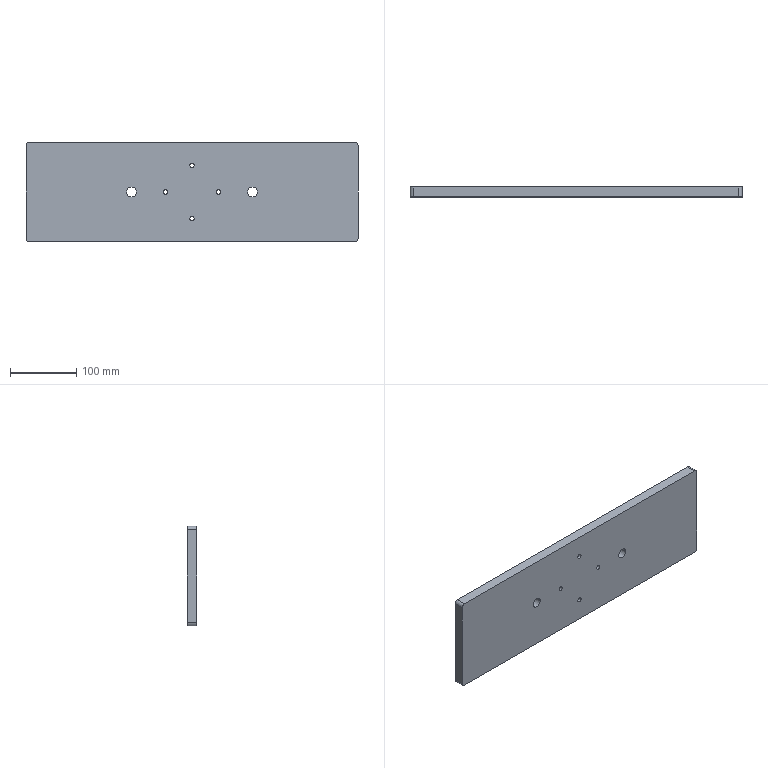Component | SolidWorks | E006TopPlate-1 | 1 solid | 22 faces | box 500 x 15 x 150 mm | volume 1117198 mm3 | cylinder 16 | plane 6 | commonest cylinder face diameters 6.8 x8 15 x4 10 x4 | material Plain Carbon Steel
build123d program:
from build123d import *

# Parameters (mm, degrees)
SKETCH1_W           = 500
SKETCH1_H           = 150
BOSS_EXTRUDE1_DEPTH = 7.5
FILLET1_R           = 5
SKETCH7_R           = 7.5
CUT_EXTRUDE2_DEPTH  = 262.438
M8_TAPPED_HOLE1_D   = 6.8


with BuildPart() as part:
    # Sketch1 → Boss-Extrude1 (new, symmetric)
    with BuildSketch(Plane.XY):
        Rectangle(SKETCH1_W, SKETCH1_H)
    extrude(amount=BOSS_EXTRUDE1_DEPTH, both=True)

    # Fillet1
    fillet1_edges = [part.edges().sort_by_distance(p)[0] for p in [
        (250, -75, 0),
        (-250, -75, 0),
        (-250, 75, 0),
        (250, 75, 0),
    ]]
    fillet(fillet1_edges, radius=FILLET1_R)

    # Sketch7 → Cut-Extrude2 (cut, through all)
    with BuildSketch(Plane.XY.offset(7.5)):
        with Locations((-91, 0)):
            Circle(SKETCH7_R)
    cut_extrude2 = extrude(amount=-CUT_EXTRUDE2_DEPTH, mode=Mode.SUBTRACT)

    # M8 Tapped Hole1 (through all)
    with Locations(Plane.XY.offset(7.5)):
        with Locations((0, 40), (0, -40), (-40, 0), (40, 0)):
            Hole(M8_TAPPED_HOLE1_D / 2)

    # Mirror1: Cut-Extrude2 across plane
    add(cut_extrude2.mirror(Plane(origin=(0, 0, 0), x_dir=(0, 0, 1), z_dir=(1, 0, 0))), mode=Mode.SUBTRACT)


solid = part.part

# Placed as in the assembly
solid = solid.moved(Location((0, 288.5, 0), (90, 0, 0)))
STEP:
#1=COLOUR_RGB('',0.7922,0.8196,0.9333);
#2=FILL_AREA_STYLE_COLOUR('',#1);
#3=FILL_AREA_STYLE('',(#2));
#4=SURFACE_STYLE_FILL_AREA(#3);
#5=SURFACE_SIDE_STYLE('',(#4));
#6=SURFACE_STYLE_USAGE(.BOTH.,#5);
#7=PRESENTATION_STYLE_ASSIGNMENT((#6));
#8=CARTESIAN_POINT('',(3.878,11.063,-0.));
#9=VERTEX_POINT('',#8);
#10=CARTESIAN_POINT('',(3.287,11.063,-0.));
#11=VERTEX_POINT('',#10);
#12=CARTESIAN_POINT('',(3.583,11.063,-0.));
#13=DIRECTION('',(0.,-1.,0.));
#14=DIRECTION('',(-1.,0.,0.));
#15=AXIS2_PLACEMENT_3D('',#12,#13,#14);
#16=CIRCLE('',#15,0.2953);
#17=EDGE_CURVE('',#9,#11,#16,.T.);
#18=ORIENTED_EDGE('',*,*,#17,.T.);
#19=CARTESIAN_POINT('',(3.287,11.654,-0.));
#20=VERTEX_POINT('',#19);
#21=CARTESIAN_POINT('',(3.287,11.063,-0.));
#22=DIRECTION('',(0.,1.,0.));
#23=VECTOR('',#22,39.37);
#24=LINE('',#21,#23);
#25=EDGE_CURVE('',#11,#20,#24,.T.);
#26=ORIENTED_EDGE('',*,*,#25,.T.);
#27=CARTESIAN_POINT('',(3.878,11.654,-0.));
#28=VERTEX_POINT('',#27);
#29=CARTESIAN_POINT('',(3.583,11.654,-0.));
#30=DIRECTION('',(0.,-1.,0.));
#31=DIRECTION('',(-1.,0.,0.));
#32=AXIS2_PLACEMENT_3D('',#29,#30,#31);
#33=CIRCLE('',#32,0.2953);
#34=EDGE_CURVE('',#28,#20,#33,.T.);
#35=ORIENTED_EDGE('',*,*,#34,.F.);
#36=CARTESIAN_POINT('',(3.878,11.063,-0.));
#37=DIRECTION('',(0.,1.,0.));
#38=VECTOR('',#37,39.37);
#39=LINE('',#36,#38);
#40=EDGE_CURVE('',#9,#28,#39,.T.);
#41=ORIENTED_EDGE('',*,*,#40,.F.);
#42=EDGE_LOOP('',(#18,#26,#35,#41));
#43=FACE_OUTER_BOUND('',#42,.T.);
#44=CARTESIAN_POINT('',(3.583,11.063,-0.));
#45=DIRECTION('',(0.,1.,0.));
#46=DIRECTION('',(1.,0.,-0.));
#47=AXIS2_PLACEMENT_3D('',#44,#45,#46);
#48=CYLINDRICAL_SURFACE('',#47,0.2953);
#49=ADVANCED_FACE('',(#43),#48,.F.);
#50=CARTESIAN_POINT('',(-0.1339,11.063,-1.575));
#51=VERTEX_POINT('',#50);
#52=CARTESIAN_POINT('',(0.1339,11.063,-1.575));
#53=VERTEX_POINT('',#52);
#54=CARTESIAN_POINT('',(-0.,11.063,-1.575));
#55=DIRECTION('',(0.,1.,0.));
#56=DIRECTION('',(1.,0.,0.));
#57=AXIS2_PLACEMENT_3D('',#54,#55,#56);
#58=CIRCLE('',#57,0.1339);
#59=EDGE_CURVE('',#51,#53,#58,.T.);
#60=ORIENTED_EDGE('',*,*,#59,.F.);
#61=CARTESIAN_POINT('',(-0.1339,11.654,-1.575));
#62=VERTEX_POINT('',#61);
#63=CARTESIAN_POINT('',(-0.1339,11.654,-1.575));
#64=DIRECTION('',(0.,1.,0.));
#65=VECTOR('',#64,39.37);
#66=LINE('',#63,#65);
#67=EDGE_CURVE('',#51,#62,#66,.T.);
#68=ORIENTED_EDGE('',*,*,#67,.T.);
#69=CARTESIAN_POINT('',(0.1339,11.654,-1.575));
#70=VERTEX_POINT('',#69);
#71=CARTESIAN_POINT('',(-0.,11.654,-1.575));
#72=DIRECTION('',(0.,1.,0.));
#73=DIRECTION('',(1.,0.,0.));
#74=AXIS2_PLACEMENT_3D('',#71,#72,#73);
#75=CIRCLE('',#74,0.1339);
#76=EDGE_CURVE('',#62,#70,#75,.T.);
#77=ORIENTED_EDGE('',*,*,#76,.T.);
#78=CARTESIAN_POINT('',(0.1339,11.654,-1.575));
#79=DIRECTION('',(0.,1.,0.));
#80=VECTOR('',#79,39.37);
#81=LINE('',#78,#80);
#82=EDGE_CURVE('',#53,#70,#81,.T.);
#83=ORIENTED_EDGE('',*,*,#82,.F.);
#84=EDGE_LOOP('',(#60,#68,#77,#83));
#85=FACE_OUTER_BOUND('',#84,.T.);
#86=CARTESIAN_POINT('',(-0.,11.654,-1.575));
#87=DIRECTION('',(0.,1.,0.));
#88=DIRECTION('',(1.,0.,0.));
#89=AXIS2_PLACEMENT_3D('',#86,#87,#88);
#90=CYLINDRICAL_SURFACE('',#89,0.1339);
#91=ADVANCED_FACE('',(#85),#90,.F.);
#92=CARTESIAN_POINT('',(-0.1339,11.063,1.575));
#93=VERTEX_POINT('',#92);
#94=CARTESIAN_POINT('',(0.1339,11.063,1.575));
#95=VERTEX_POINT('',#94);
#96=CARTESIAN_POINT('',(-0.,11.063,1.575));
#97=DIRECTION('',(0.,1.,0.));
#98=DIRECTION('',(1.,0.,0.));
#99=AXIS2_PLACEMENT_3D('',#96,#97,#98);
#100=CIRCLE('',#99,0.1339);
#101=EDGE_CURVE('',#93,#95,#100,.T.);
#102=ORIENTED_EDGE('',*,*,#101,.F.);
#103=CARTESIAN_POINT('',(-0.1339,11.654,1.575));
#104=VERTEX_POINT('',#103);
#105=CARTESIAN_POINT('',(-0.1339,11.654,1.575));
#106=DIRECTION('',(0.,1.,0.));
#107=VECTOR('',#106,39.37);
#108=LINE('',#105,#107);
#109=EDGE_CURVE('',#93,#104,#108,.T.);
#110=ORIENTED_EDGE('',*,*,#109,.T.);
#111=CARTESIAN_POINT('',(0.1339,11.654,1.575));
#112=VERTEX_POINT('',#111);
#113=CARTESIAN_POINT('',(-0.,11.654,1.575));
#114=DIRECTION('',(0.,1.,0.));
#115=DIRECTION('',(1.,0.,0.));
#116=AXIS2_PLACEMENT_3D('',#113,#114,#115);
#117=CIRCLE('',#116,0.1339);
#118=EDGE_CURVE('',#104,#112,#117,.T.);
#119=ORIENTED_EDGE('',*,*,#118,.T.);
#120=CARTESIAN_POINT('',(0.1339,11.654,1.575));
#121=DIRECTION('',(0.,1.,0.));
#122=VECTOR('',#121,39.37);
#123=LINE('',#120,#122);
#124=EDGE_CURVE('',#95,#112,#123,.T.);
#125=ORIENTED_EDGE('',*,*,#124,.F.);
#126=EDGE_LOOP('',(#102,#110,#119,#125));
#127=FACE_OUTER_BOUND('',#126,.T.);
#128=CARTESIAN_POINT('',(-0.,11.654,1.575));
#129=DIRECTION('',(0.,1.,0.));
#130=DIRECTION('',(1.,0.,0.));
#131=AXIS2_PLACEMENT_3D('',#128,#129,#130);
#132=CYLINDRICAL_SURFACE('',#131,0.1339);
#133=ADVANCED_FACE('',(#127),#132,.F.);
#134=CARTESIAN_POINT('',(-1.709,11.063,0.));
#135=VERTEX_POINT('',#134);
#136=CARTESIAN_POINT('',(-1.441,11.063,0.));
#137=VERTEX_POINT('',#136);
#138=CARTESIAN_POINT('',(-1.575,11.063,0.));
#139=DIRECTION('',(0.,1.,0.));
#140=DIRECTION('',(1.,0.,-0.));
#141=AXIS2_PLACEMENT_3D('',#138,#139,#140);
#142=CIRCLE('',#141,0.1339);
#143=EDGE_CURVE('',#135,#137,#142,.T.);
#144=ORIENTED_EDGE('',*,*,#143,.F.);
#145=CARTESIAN_POINT('',(-1.709,11.654,0.));
#146=VERTEX_POINT('',#145);
#147=CARTESIAN_POINT('',(-1.709,11.654,0.));
#148=DIRECTION('',(0.,1.,0.));
#149=VECTOR('',#148,39.37);
#150=LINE('',#147,#149);
#151=EDGE_CURVE('',#135,#146,#150,.T.);
#152=ORIENTED_EDGE('',*,*,#151,.T.);
#153=CARTESIAN_POINT('',(-1.441,11.654,0.));
#154=VERTEX_POINT('',#153);
#155=CARTESIAN_POINT('',(-1.575,11.654,0.));
#156=DIRECTION('',(0.,1.,0.));
#157=DIRECTION('',(1.,0.,-0.));
#158=AXIS2_PLACEMENT_3D('',#155,#156,#157);
#159=CIRCLE('',#158,0.1339);
#160=EDGE_CURVE('',#146,#154,#159,.T.);
#161=ORIENTED_EDGE('',*,*,#160,.T.);
#162=CARTESIAN_POINT('',(-1.441,11.654,0.));
#163=DIRECTION('',(0.,1.,0.));
#164=VECTOR('',#163,39.37);
#165=LINE('',#162,#164);
#166=EDGE_CURVE('',#137,#154,#165,.T.);
#167=ORIENTED_EDGE('',*,*,#166,.F.);
#168=EDGE_LOOP('',(#144,#152,#161,#167));
#169=FACE_OUTER_BOUND('',#168,.T.);
#170=CARTESIAN_POINT('',(-1.575,11.654,0.));
#171=DIRECTION('',(0.,1.,0.));
#172=DIRECTION('',(1.,0.,-0.));
#173=AXIS2_PLACEMENT_3D('',#170,#171,#172);
#174=CYLINDRICAL_SURFACE('',#173,0.1339);
#175=ADVANCED_FACE('',(#169),#174,.F.);
#176=CARTESIAN_POINT('',(1.441,11.063,-0.));
#177=VERTEX_POINT('',#176);
#178=CARTESIAN_POINT('',(1.709,11.063,0.));
#179=VERTEX_POINT('',#178);
#180=CARTESIAN_POINT('',(1.575,11.063,0.));
#181=DIRECTION('',(0.,1.,0.));
#182=DIRECTION('',(1.,0.,-0.));
#183=AXIS2_PLACEMENT_3D('',#180,#181,#182);
#184=CIRCLE('',#183,0.1339);
#185=EDGE_CURVE('',#177,#179,#184,.T.);
#186=ORIENTED_EDGE('',*,*,#185,.F.);
#187=CARTESIAN_POINT('',(1.441,11.654,-0.));
#188=VERTEX_POINT('',#187);
#189=CARTESIAN_POINT('',(1.441,11.654,-0.));
#190=DIRECTION('',(0.,1.,0.));
#191=VECTOR('',#190,39.37);
#192=LINE('',#189,#191);
#193=EDGE_CURVE('',#177,#188,#192,.T.);
#194=ORIENTED_EDGE('',*,*,#193,.T.);
#195=CARTESIAN_POINT('',(1.709,11.654,0.));
#196=VERTEX_POINT('',#195);
#197=CARTESIAN_POINT('',(1.575,11.654,0.));
#198=DIRECTION('',(0.,1.,0.));
#199=DIRECTION('',(1.,0.,-0.));
#200=AXIS2_PLACEMENT_3D('',#197,#198,#199);
#201=CIRCLE('',#200,0.1339);
#202=EDGE_CURVE('',#188,#196,#201,.T.);
#203=ORIENTED_EDGE('',*,*,#202,.T.);
#204=CARTESIAN_POINT('',(1.709,11.654,0.));
#205=DIRECTION('',(0.,1.,0.));
#206=VECTOR('',#205,39.37);
#207=LINE('',#204,#206);
#208=EDGE_CURVE('',#179,#196,#207,.T.);
#209=ORIENTED_EDGE('',*,*,#208,.F.);
#210=EDGE_LOOP('',(#186,#194,#203,#209));
#211=FACE_OUTER_BOUND('',#210,.T.);
#212=CARTESIAN_POINT('',(1.575,11.654,0.));
#213=DIRECTION('',(0.,1.,0.));
#214=DIRECTION('',(1.,0.,-0.));
#215=AXIS2_PLACEMENT_3D('',#212,#213,#214);
#216=CYLINDRICAL_SURFACE('',#215,0.1339);
#217=ADVANCED_FACE('',(#211),#216,.F.);
#218=CARTESIAN_POINT('',(-3.878,11.063,0.));
#219=VERTEX_POINT('',#218);
#220=CARTESIAN_POINT('',(-3.287,11.063,0.));
#221=VERTEX_POINT('',#220);
#222=CARTESIAN_POINT('',(-3.583,11.063,0.));
#223=DIRECTION('',(0.,1.,0.));
#224=DIRECTION('',(1.,0.,-0.));
#225=AXIS2_PLACEMENT_3D('',#222,#223,#224);
#226=CIRCLE('',#225,0.2953);
#227=EDGE_CURVE('',#219,#221,#226,.T.);
#228=ORIENTED_EDGE('',*,*,#227,.F.);
#229=CARTESIAN_POINT('',(-3.878,11.654,0.));
#230=VERTEX_POINT('',#229);
#231=CARTESIAN_POINT('',(-3.878,11.063,0.));
#232=DIRECTION('',(0.,1.,0.));
#233=VECTOR('',#232,39.37);
#234=LINE('',#231,#233);
#235=EDGE_CURVE('',#219,#230,#234,.T.);
#236=ORIENTED_EDGE('',*,*,#235,.T.);
#237=CARTESIAN_POINT('',(-3.287,11.654,0.));
#238=VERTEX_POINT('',#237);
#239=CARTESIAN_POINT('',(-3.583,11.654,0.));
#240=DIRECTION('',(0.,1.,0.));
#241=DIRECTION('',(1.,0.,-0.));
#242=AXIS2_PLACEMENT_3D('',#239,#240,#241);
#243=CIRCLE('',#242,0.2953);
#244=EDGE_CURVE('',#230,#238,#243,.T.);
#245=ORIENTED_EDGE('',*,*,#244,.T.);
#246=CARTESIAN_POINT('',(-3.287,11.063,0.));
#247=DIRECTION('',(0.,1.,0.));
#248=VECTOR('',#247,39.37);
#249=LINE('',#246,#248);
#250=EDGE_CURVE('',#221,#238,#249,.T.);
#251=ORIENTED_EDGE('',*,*,#250,.F.);
#252=EDGE_LOOP('',(#228,#236,#245,#251));
#253=FACE_OUTER_BOUND('',#252,.T.);
#254=CARTESIAN_POINT('',(-3.583,11.063,0.));
#255=DIRECTION('',(0.,1.,0.));
#256=DIRECTION('',(1.,0.,-0.));
#257=AXIS2_PLACEMENT_3D('',#254,#255,#256);
#258=CYLINDRICAL_SURFACE('',#257,0.2953);
#259=ADVANCED_FACE('',(#253),#258,.F.);
#260=CARTESIAN_POINT('',(-9.646,11.654,2.953));
#261=VERTEX_POINT('',#260);
#262=CARTESIAN_POINT('',(9.646,11.654,2.953));
#263=VERTEX_POINT('',#262);
#264=CARTESIAN_POINT('',(-9.843,11.654,2.953));
#265=DIRECTION('',(1.,0.,-0.));
#266=VECTOR('',#265,39.37);
#267=LINE('',#264,#266);
#268=EDGE_CURVE('',#261,#263,#267,.T.);
#269=ORIENTED_EDGE('',*,*,#268,.T.);
#270=CARTESIAN_POINT('',(9.843,11.654,2.756));
#271=VERTEX_POINT('',#270);
#272=CARTESIAN_POINT('',(9.646,11.654,2.756));
#273=DIRECTION('',(0.,1.,0.));
#274=DIRECTION('',(1.,0.,0.));
#275=AXIS2_PLACEMENT_3D('',#272,#273,#274);
#276=CIRCLE('',#275,0.1969);
#277=EDGE_CURVE('',#263,#271,#276,.T.);
#278=ORIENTED_EDGE('',*,*,#277,.T.);
#279=CARTESIAN_POINT('',(9.843,11.654,-2.756));
#280=VERTEX_POINT('',#279);
#281=CARTESIAN_POINT('',(9.843,11.654,-2.953));
#282=DIRECTION('',(-0.,0.,-1.));
#283=VECTOR('',#282,39.37);
#284=LINE('',#281,#283);
#285=EDGE_CURVE('',#271,#280,#284,.T.);
#286=ORIENTED_EDGE('',*,*,#285,.T.);
#287=CARTESIAN_POINT('',(9.646,11.654,-2.953));
#288=VERTEX_POINT('',#287);
#289=CARTESIAN_POINT('',(9.646,11.654,-2.756));
#290=DIRECTION('',(0.,1.,0.));
#291=DIRECTION('',(1.,0.,0.));
#292=AXIS2_PLACEMENT_3D('',#289,#290,#291);
#293=CIRCLE('',#292,0.1969);
#294=EDGE_CURVE('',#280,#288,#293,.T.);
#295=ORIENTED_EDGE('',*,*,#294,.T.);
#296=CARTESIAN_POINT('',(-9.646,11.654,-2.953));
#297=VERTEX_POINT('',#296);
#298=CARTESIAN_POINT('',(-9.843,11.654,-2.953));
#299=DIRECTION('',(-1.,0.,0.));
#300=VECTOR('',#299,39.37);
#301=LINE('',#298,#300);
#302=EDGE_CURVE('',#288,#297,#301,.T.);
#303=ORIENTED_EDGE('',*,*,#302,.T.);
#304=CARTESIAN_POINT('',(-9.843,11.654,-2.756));
#305=VERTEX_POINT('',#304);
#306=CARTESIAN_POINT('',(-9.646,11.654,-2.756));
#307=DIRECTION('',(0.,1.,0.));
#308=DIRECTION('',(1.,0.,0.));
#309=AXIS2_PLACEMENT_3D('',#306,#307,#308);
#310=CIRCLE('',#309,0.1969);
#311=EDGE_CURVE('',#297,#305,#310,.T.);
#312=ORIENTED_EDGE('',*,*,#311,.T.);
#313=CARTESIAN_POINT('',(-9.843,11.654,2.756));
#314=VERTEX_POINT('',#313);
#315=CARTESIAN_POINT('',(-9.843,11.654,-2.953));
#316=DIRECTION('',(0.,0.,1.));
#317=VECTOR('',#316,39.37);
#318=LINE('',#315,#317);
#319=EDGE_CURVE('',#305,#314,#318,.T.);
#320=ORIENTED_EDGE('',*,*,#319,.T.);
#321=CARTESIAN_POINT('',(-9.646,11.654,2.756));
#322=DIRECTION('',(0.,1.,0.));
#323=DIRECTION('',(1.,0.,0.));
#324=AXIS2_PLACEMENT_3D('',#321,#322,#323);
#325=CIRCLE('',#324,0.1969);
#326=EDGE_CURVE('',#314,#261,#325,.T.);
#327=ORIENTED_EDGE('',*,*,#326,.T.);
#328=EDGE_LOOP('',(#269,#278,#286,#295,#303,#312,#320,#327));
#329=FACE_OUTER_BOUND('',#328,.T.);
#330=CARTESIAN_POINT('',(-3.583,11.654,0.));
#331=DIRECTION('',(0.,1.,0.));
#332=DIRECTION('',(1.,0.,-0.));
#333=AXIS2_PLACEMENT_3D('',#330,#331,#332);
#334=CIRCLE('',#333,0.2953);
#335=EDGE_CURVE('',#238,#230,#334,.T.);
#336=ORIENTED_EDGE('',*,*,#335,.F.);
#337=ORIENTED_EDGE('',*,*,#244,.F.);
#338=EDGE_LOOP('',(#336,#337));
#339=FACE_BOUND('',#338,.T.);
#340=CARTESIAN_POINT('',(1.575,11.654,0.));
#341=DIRECTION('',(0.,1.,0.));
#342=DIRECTION('',(1.,0.,-0.));
#343=AXIS2_PLACEMENT_3D('',#340,#341,#342);
#344=CIRCLE('',#343,0.1339);
#345=EDGE_CURVE('',#196,#188,#344,.T.);
#346=ORIENTED_EDGE('',*,*,#345,.F.);
#347=ORIENTED_EDGE('',*,*,#202,.F.);
#348=EDGE_LOOP('',(#346,#347));
#349=FACE_BOUND('',#348,.T.);
#350=CARTESIAN_POINT('',(-1.575,11.654,0.));
#351=DIRECTION('',(0.,1.,0.));
#352=DIRECTION('',(1.,0.,-0.));
#353=AXIS2_PLACEMENT_3D('',#350,#351,#352);
#354=CIRCLE('',#353,0.1339);
#355=EDGE_CURVE('',#154,#146,#354,.T.);
#356=ORIENTED_EDGE('',*,*,#355,.F.);
#357=ORIENTED_EDGE('',*,*,#160,.F.);
#358=EDGE_LOOP('',(#356,#357));
#359=FACE_BOUND('',#358,.T.);
#360=CARTESIAN_POINT('',(-0.,11.654,1.575));
#361=DIRECTION('',(0.,1.,0.));
#362=DIRECTION('',(1.,0.,0.));
#363=AXIS2_PLACEMENT_3D('',#360,#361,#362);
#364=CIRCLE('',#363,0.1339);
#365=EDGE_CURVE('',#112,#104,#364,.T.);
#366=ORIENTED_EDGE('',*,*,#365,.F.);
#367=ORIENTED_EDGE('',*,*,#118,.F.);
#368=EDGE_LOOP('',(#366,#367));
#369=FACE_BOUND('',#368,.T.);
#370=CARTESIAN_POINT('',(-0.,11.654,-1.575));
#371=DIRECTION('',(0.,1.,0.));
#372=DIRECTION('',(1.,0.,0.));
#373=AXIS2_PLACEMENT_3D('',#370,#371,#372);
#374=CIRCLE('',#373,0.1339);
#375=EDGE_CURVE('',#70,#62,#374,.T.);
#376=ORIENTED_EDGE('',*,*,#375,.F.);
#377=ORIENTED_EDGE('',*,*,#76,.F.);
#378=EDGE_LOOP('',(#376,#377));
#379=FACE_BOUND('',#378,.T.);
#380=ORIENTED_EDGE('',*,*,#34,.T.);
#381=CARTESIAN_POINT('',(3.583,11.654,-0.));
#382=DIRECTION('',(0.,-1.,0.));
#383=DIRECTION('',(-1.,0.,0.));
#384=AXIS2_PLACEMENT_3D('',#381,#382,#383);
#385=CIRCLE('',#384,0.2953);
#386=EDGE_CURVE('',#20,#28,#385,.T.);
#387=ORIENTED_EDGE('',*,*,#386,.T.);
#388=EDGE_LOOP('',(#380,#387));
#389=FACE_BOUND('',#388,.T.);
#390=CARTESIAN_POINT('',(9.843,11.654,2.953));
#391=DIRECTION('',(0.,1.,0.));
#392=DIRECTION('',(1.,0.,-0.));
#393=AXIS2_PLACEMENT_3D('',#390,#391,#392);
#394=PLANE('',#393);
#395=ADVANCED_FACE('',(#329,#339,#349,#359,#369,#379,#389),#394,.T.);
#396=CARTESIAN_POINT('',(9.843,11.063,2.756));
#397=VERTEX_POINT('',#396);
#398=CARTESIAN_POINT('',(9.843,11.063,-2.756));
#399=VERTEX_POINT('',#398);
#400=CARTESIAN_POINT('',(9.843,11.063,-2.953));
#401=DIRECTION('',(-0.,0.,-1.));
#402=VECTOR('',#401,39.37);
#403=LINE('',#400,#402);
#404=EDGE_CURVE('',#397,#399,#403,.T.);
#405=ORIENTED_EDGE('',*,*,#404,.F.);
#406=CARTESIAN_POINT('',(9.646,11.063,2.953));
#407=VERTEX_POINT('',#406);
#408=CARTESIAN_POINT('',(9.646,11.063,2.756));
#409=DIRECTION('',(0.,-1.,0.));
#410=DIRECTION('',(1.,0.,0.));
#411=AXIS2_PLACEMENT_3D('',#408,#409,#410);
#412=CIRCLE('',#411,0.1969);
#413=EDGE_CURVE('',#397,#407,#412,.T.);
#414=ORIENTED_EDGE('',*,*,#413,.T.);
#415=CARTESIAN_POINT('',(-9.646,11.063,2.953));
#416=VERTEX_POINT('',#415);
#417=CARTESIAN_POINT('',(-9.843,11.063,2.953));
#418=DIRECTION('',(1.,0.,-0.));
#419=VECTOR('',#418,39.37);
#420=LINE('',#417,#419);
#421=EDGE_CURVE('',#416,#407,#420,.T.);
#422=ORIENTED_EDGE('',*,*,#421,.F.);
#423=CARTESIAN_POINT('',(-9.843,11.063,2.756));
#424=VERTEX_POINT('',#423);
#425=CARTESIAN_POINT('',(-9.646,11.063,2.756));
#426=DIRECTION('',(0.,-1.,0.));
#427=DIRECTION('',(1.,0.,0.));
#428=AXIS2_PLACEMENT_3D('',#425,#426,#427);
#429=CIRCLE('',#428,0.1969);
#430=EDGE_CURVE('',#416,#424,#429,.T.);
#431=ORIENTED_EDGE('',*,*,#430,.T.);
#432=CARTESIAN_POINT('',(-9.843,11.063,-2.756));
#433=VERTEX_POINT('',#432);
#434=CARTESIAN_POINT('',(-9.843,11.063,-2.953));
#435=DIRECTION('',(0.,0.,1.));
#436=VECTOR('',#435,39.37);
#437=LINE('',#434,#436);
#438=EDGE_CURVE('',#433,#424,#437,.T.);
#439=ORIENTED_EDGE('',*,*,#438,.F.);
#440=CARTESIAN_POINT('',(-9.646,11.063,-2.953));
#441=VERTEX_POINT('',#440);
#442=CARTESIAN_POINT('',(-9.646,11.063,-2.756));
#443=DIRECTION('',(0.,-1.,0.));
#444=DIRECTION('',(1.,0.,0.));
#445=AXIS2_PLACEMENT_3D('',#442,#443,#444);
#446=CIRCLE('',#445,0.1969);
#447=EDGE_CURVE('',#433,#441,#446,.T.);
#448=ORIENTED_EDGE('',*,*,#447,.T.);
#449=CARTESIAN_POINT('',(9.646,11.063,-2.953));
#450=VERTEX_POINT('',#449);
#451=CARTESIAN_POINT('',(-9.843,11.063,-2.953));
#452=DIRECTION('',(-1.,0.,0.));
#453=VECTOR('',#452,39.37);
#454=LINE('',#451,#453);
#455=EDGE_CURVE('',#450,#441,#454,.T.);
#456=ORIENTED_EDGE('',*,*,#455,.F.);
#457=CARTESIAN_POINT('',(9.646,11.063,-2.756));
#458=DIRECTION('',(0.,-1.,0.));
#459=DIRECTION('',(1.,0.,0.));
#460=AXIS2_PLACEMENT_3D('',#457,#458,#459);
#461=CIRCLE('',#460,0.1969);
#462=EDGE_CURVE('',#450,#399,#461,.T.);
#463=ORIENTED_EDGE('',*,*,#462,.T.);
#464=EDGE_LOOP('',(#405,#414,#422,#431,#439,#448,#456,#463));
#465=FACE_OUTER_BOUND('',#464,.T.);
#466=CARTESIAN_POINT('',(-3.583,11.063,0.));
#467=DIRECTION('',(0.,1.,0.));
#468=DIRECTION('',(1.,0.,-0.));
#469=AXIS2_PLACEMENT_3D('',#466,#467,#468);
#470=CIRCLE('',#469,0.2953);
#471=EDGE_CURVE('',#221,#219,#470,.T.);
#472=ORIENTED_EDGE('',*,*,#471,.T.);
#473=ORIENTED_EDGE('',*,*,#227,.T.);
#474=EDGE_LOOP('',(#472,#473));
#475=FACE_BOUND('',#474,.T.);
#476=CARTESIAN_POINT('',(1.575,11.063,0.));
#477=DIRECTION('',(0.,1.,0.));
#478=DIRECTION('',(1.,0.,-0.));
#479=AXIS2_PLACEMENT_3D('',#476,#477,#478);
#480=CIRCLE('',#479,0.1339);
#481=EDGE_CURVE('',#179,#177,#480,.T.);
#482=ORIENTED_EDGE('',*,*,#481,.T.);
#483=ORIENTED_EDGE('',*,*,#185,.T.);
#484=EDGE_LOOP('',(#482,#483));
#485=FACE_BOUND('',#484,.T.);
#486=CARTESIAN_POINT('',(-1.575,11.063,0.));
#487=DIRECTION('',(0.,1.,0.));
#488=DIRECTION('',(1.,0.,-0.));
#489=AXIS2_PLACEMENT_3D('',#486,#487,#488);
#490=CIRCLE('',#489,0.1339);
#491=EDGE_CURVE('',#137,#135,#490,.T.);
#492=ORIENTED_EDGE('',*,*,#491,.T.);
#493=ORIENTED_EDGE('',*,*,#143,.T.);
#494=EDGE_LOOP('',(#492,#493));
#495=FACE_BOUND('',#494,.T.);
#496=CARTESIAN_POINT('',(-0.,11.063,1.575));
#497=DIRECTION('',(0.,1.,0.));
#498=DIRECTION('',(1.,0.,0.));
#499=AXIS2_PLACEMENT_3D('',#496,#497,#498);
#500=CIRCLE('',#499,0.1339);
#501=EDGE_CURVE('',#95,#93,#500,.T.);
#502=ORIENTED_EDGE('',*,*,#501,.T.);
#503=ORIENTED_EDGE('',*,*,#101,.T.);
#504=EDGE_LOOP('',(#502,#503));
#505=FACE_BOUND('',#504,.T.);
#506=CARTESIAN_POINT('',(-0.,11.063,-1.575));
#507=DIRECTION('',(0.,1.,0.));
#508=DIRECTION('',(1.,0.,0.));
#509=AXIS2_PLACEMENT_3D('',#506,#507,#508);
#510=CIRCLE('',#509,0.1339);
#511=EDGE_CURVE('',#53,#51,#510,.T.);
#512=ORIENTED_EDGE('',*,*,#511,.T.);
#513=ORIENTED_EDGE('',*,*,#59,.T.);
#514=EDGE_LOOP('',(#512,#513));
#515=FACE_BOUND('',#514,.T.);
#516=ORIENTED_EDGE('',*,*,#17,.F.);
#517=CARTESIAN_POINT('',(3.583,11.063,-0.));
#518=DIRECTION('',(0.,-1.,0.));
#519=DIRECTION('',(-1.,0.,0.));
#520=AXIS2_PLACEMENT_3D('',#517,#518,#519);
#521=CIRCLE('',#520,0.2953);
#522=EDGE_CURVE('',#11,#9,#521,.T.);
#523=ORIENTED_EDGE('',*,*,#522,.F.);
#524=EDGE_LOOP('',(#516,#523));
#525=FACE_BOUND('',#524,.T.);
#526=CARTESIAN_POINT('',(9.843,11.063,2.953));
#527=DIRECTION('',(0.,1.,0.));
#528=DIRECTION('',(1.,0.,-0.));
#529=AXIS2_PLACEMENT_3D('',#526,#527,#528);
#530=PLANE('',#529);
#531=ADVANCED_FACE('',(#465,#475,#485,#495,#505,#515,#525),#530,.F.);
#532=ORIENTED_EDGE('',*,*,#285,.F.);
#533=CARTESIAN_POINT('',(9.843,11.654,2.756));
#534=DIRECTION('',(0.,-1.,0.));
#535=VECTOR('',#534,39.37);
#536=LINE('',#533,#535);
#537=EDGE_CURVE('',#271,#397,#536,.T.);
#538=ORIENTED_EDGE('',*,*,#537,.T.);
#539=ORIENTED_EDGE('',*,*,#404,.T.);
#540=CARTESIAN_POINT('',(9.843,11.654,-2.756));
#541=DIRECTION('',(0.,1.,0.));
#542=VECTOR('',#541,39.37);
#543=LINE('',#540,#542);
#544=EDGE_CURVE('',#399,#280,#543,.T.);
#545=ORIENTED_EDGE('',*,*,#544,.T.);
#546=EDGE_LOOP('',(#532,#538,#539,#545));
#547=FACE_OUTER_BOUND('',#546,.T.);
#548=CARTESIAN_POINT('',(9.843,11.654,-2.953));
#549=DIRECTION('',(-1.,0.,0.));
#550=DIRECTION('',(0.,0.,1.));
#551=AXIS2_PLACEMENT_3D('',#548,#549,#550);
#552=PLANE('',#551);
#553=ADVANCED_FACE('',(#547),#552,.F.);
#554=ORIENTED_EDGE('',*,*,#455,.T.);
#555=CARTESIAN_POINT('',(-9.646,11.654,-2.953));
#556=DIRECTION('',(0.,1.,0.));
#557=VECTOR('',#556,39.37);
#558=LINE('',#555,#557);
#559=EDGE_CURVE('',#441,#297,#558,.T.);
#560=ORIENTED_EDGE('',*,*,#559,.T.);
#561=ORIENTED_EDGE('',*,*,#302,.F.);
#562=CARTESIAN_POINT('',(9.646,11.654,-2.953));
#563=DIRECTION('',(0.,-1.,0.));
#564=VECTOR('',#563,39.37);
#565=LINE('',#562,#564);
#566=EDGE_CURVE('',#288,#450,#565,.T.);
#567=ORIENTED_EDGE('',*,*,#566,.T.);
#568=EDGE_LOOP('',(#554,#560,#561,#567));
#569=FACE_OUTER_BOUND('',#568,.T.);
#570=CARTESIAN_POINT('',(-9.843,11.654,-2.953));
#571=DIRECTION('',(0.,0.,1.));
#572=DIRECTION('',(0.,-1.,0.));
#573=AXIS2_PLACEMENT_3D('',#570,#571,#572);
#574=PLANE('',#573);
#575=ADVANCED_FACE('',(#569),#574,.F.);
#576=ORIENTED_EDGE('',*,*,#438,.T.);
#577=CARTESIAN_POINT('',(-9.843,11.654,2.756));
#578=DIRECTION('',(0.,1.,0.));
#579=VECTOR('',#578,39.37);
#580=LINE('',#577,#579);
#581=EDGE_CURVE('',#424,#314,#580,.T.);
#582=ORIENTED_EDGE('',*,*,#581,.T.);
#583=ORIENTED_EDGE('',*,*,#319,.F.);
#584=CARTESIAN_POINT('',(-9.843,11.654,-2.756));
#585=DIRECTION('',(0.,-1.,0.));
#586=VECTOR('',#585,39.37);
#587=LINE('',#584,#586);
#588=EDGE_CURVE('',#305,#433,#587,.T.);
#589=ORIENTED_EDGE('',*,*,#588,.T.);
#590=EDGE_LOOP('',(#576,#582,#583,#589));
#591=FACE_OUTER_BOUND('',#590,.T.);
#592=CARTESIAN_POINT('',(-9.843,11.654,-2.953));
#593=DIRECTION('',(1.,0.,-0.));
#594=DIRECTION('',(0.,-1.,0.));
#595=AXIS2_PLACEMENT_3D('',#592,#593,#594);
#596=PLANE('',#595);
#597=ADVANCED_FACE('',(#591),#596,.F.);
#598=ORIENTED_EDGE('',*,*,#421,.T.);
#599=CARTESIAN_POINT('',(9.646,11.654,2.953));
#600=DIRECTION('',(0.,1.,0.));
#601=VECTOR('',#600,39.37);
#602=LINE('',#599,#601);
#603=EDGE_CURVE('',#407,#263,#602,.T.);
#604=ORIENTED_EDGE('',*,*,#603,.T.);
#605=ORIENTED_EDGE('',*,*,#268,.F.);
#606=CARTESIAN_POINT('',(-9.646,11.654,2.953));
#607=DIRECTION('',(0.,-1.,0.));
#608=VECTOR('',#607,39.37);
#609=LINE('',#606,#608);
#610=EDGE_CURVE('',#261,#416,#609,.T.);
#611=ORIENTED_EDGE('',*,*,#610,.T.);
#612=EDGE_LOOP('',(#598,#604,#605,#611));
#613=FACE_OUTER_BOUND('',#612,.T.);
#614=CARTESIAN_POINT('',(-9.843,11.654,2.953));
#615=DIRECTION('',(-0.,0.,-1.));
#616=DIRECTION('',(0.,1.,0.));
#617=AXIS2_PLACEMENT_3D('',#614,#615,#616);
#618=PLANE('',#617);
#619=ADVANCED_FACE('',(#613),#618,.F.);
#620=ORIENTED_EDGE('',*,*,#277,.F.);
#621=ORIENTED_EDGE('',*,*,#603,.F.);
#622=ORIENTED_EDGE('',*,*,#413,.F.);
#623=ORIENTED_EDGE('',*,*,#537,.F.);
#624=EDGE_LOOP('',(#620,#621,#622,#623));
#625=FACE_OUTER_BOUND('',#624,.T.);
#626=CARTESIAN_POINT('',(9.646,11.654,2.756));
#627=DIRECTION('',(0.,-1.,0.));
#628=DIRECTION('',(-1.,0.,0.));
#629=AXIS2_PLACEMENT_3D('',#626,#627,#628);
#630=CYLINDRICAL_SURFACE('',#629,0.1969);
#631=ADVANCED_FACE('',(#625),#630,.T.);
#632=ORIENTED_EDGE('',*,*,#326,.F.);
#633=ORIENTED_EDGE('',*,*,#581,.F.);
#634=ORIENTED_EDGE('',*,*,#430,.F.);
#635=ORIENTED_EDGE('',*,*,#610,.F.);
#636=EDGE_LOOP('',(#632,#633,#634,#635));
#637=FACE_OUTER_BOUND('',#636,.T.);
#638=CARTESIAN_POINT('',(-9.646,11.654,2.756));
#639=DIRECTION('',(0.,-1.,0.));
#640=DIRECTION('',(-1.,0.,0.));
#641=AXIS2_PLACEMENT_3D('',#638,#639,#640);
#642=CYLINDRICAL_SURFACE('',#641,0.1969);
#643=ADVANCED_FACE('',(#637),#642,.T.);
#644=ORIENTED_EDGE('',*,*,#311,.F.);
#645=ORIENTED_EDGE('',*,*,#559,.F.);
#646=ORIENTED_EDGE('',*,*,#447,.F.);
#647=ORIENTED_EDGE('',*,*,#588,.F.);
#648=EDGE_LOOP('',(#644,#645,#646,#647));
#649=FACE_OUTER_BOUND('',#648,.T.);
#650=CARTESIAN_POINT('',(-9.646,11.654,-2.756));
#651=DIRECTION('',(0.,-1.,0.));
#652=DIRECTION('',(-1.,0.,0.));
#653=AXIS2_PLACEMENT_3D('',#650,#651,#652);
#654=CYLINDRICAL_SURFACE('',#653,0.1969);
#655=ADVANCED_FACE('',(#649),#654,.T.);
#656=ORIENTED_EDGE('',*,*,#294,.F.);
#657=ORIENTED_EDGE('',*,*,#544,.F.);
#658=ORIENTED_EDGE('',*,*,#462,.F.);
#659=ORIENTED_EDGE('',*,*,#566,.F.);
#660=EDGE_LOOP('',(#656,#657,#658,#659));
#661=FACE_OUTER_BOUND('',#660,.T.);
#662=CARTESIAN_POINT('',(9.646,11.654,-2.756));
#663=DIRECTION('',(0.,-1.,0.));
#664=DIRECTION('',(-1.,0.,0.));
#665=AXIS2_PLACEMENT_3D('',#662,#663,#664);
#666=CYLINDRICAL_SURFACE('',#665,0.1969);
#667=ADVANCED_FACE('',(#661),#666,.T.);
#668=ORIENTED_EDGE('',*,*,#235,.F.);
#669=ORIENTED_EDGE('',*,*,#471,.F.);
#670=ORIENTED_EDGE('',*,*,#250,.T.);
#671=ORIENTED_EDGE('',*,*,#335,.T.);
#672=EDGE_LOOP('',(#668,#669,#670,#671));
#673=FACE_OUTER_BOUND('',#672,.T.);
#674=CARTESIAN_POINT('',(-3.583,11.063,0.));
#675=DIRECTION('',(0.,1.,0.));
#676=DIRECTION('',(1.,0.,-0.));
#677=AXIS2_PLACEMENT_3D('',#674,#675,#676);
#678=CYLINDRICAL_SURFACE('',#677,0.2953);
#679=ADVANCED_FACE('',(#673),#678,.F.);
#680=ORIENTED_EDGE('',*,*,#193,.F.);
#681=ORIENTED_EDGE('',*,*,#481,.F.);
#682=ORIENTED_EDGE('',*,*,#208,.T.);
#683=ORIENTED_EDGE('',*,*,#345,.T.);
#684=EDGE_LOOP('',(#680,#681,#682,#683));
#685=FACE_OUTER_BOUND('',#684,.T.);
#686=CARTESIAN_POINT('',(1.575,11.654,0.));
#687=DIRECTION('',(0.,1.,0.));
#688=DIRECTION('',(1.,0.,-0.));
#689=AXIS2_PLACEMENT_3D('',#686,#687,#688);
#690=CYLINDRICAL_SURFACE('',#689,0.1339);
#691=ADVANCED_FACE('',(#685),#690,.F.);
#692=ORIENTED_EDGE('',*,*,#151,.F.);
#693=ORIENTED_EDGE('',*,*,#491,.F.);
#694=ORIENTED_EDGE('',*,*,#166,.T.);
#695=ORIENTED_EDGE('',*,*,#355,.T.);
#696=EDGE_LOOP('',(#692,#693,#694,#695));
#697=FACE_OUTER_BOUND('',#696,.T.);
#698=CARTESIAN_POINT('',(-1.575,11.654,0.));
#699=DIRECTION('',(0.,1.,0.));
#700=DIRECTION('',(1.,0.,-0.));
#701=AXIS2_PLACEMENT_3D('',#698,#699,#700);
#702=CYLINDRICAL_SURFACE('',#701,0.1339);
#703=ADVANCED_FACE('',(#697),#702,.F.);
#704=ORIENTED_EDGE('',*,*,#109,.F.);
#705=ORIENTED_EDGE('',*,*,#501,.F.);
#706=ORIENTED_EDGE('',*,*,#124,.T.);
#707=ORIENTED_EDGE('',*,*,#365,.T.);
#708=EDGE_LOOP('',(#704,#705,#706,#707));
#709=FACE_OUTER_BOUND('',#708,.T.);
#710=CARTESIAN_POINT('',(-0.,11.654,1.575));
#711=DIRECTION('',(0.,1.,0.));
#712=DIRECTION('',(1.,0.,0.));
#713=AXIS2_PLACEMENT_3D('',#710,#711,#712);
#714=CYLINDRICAL_SURFACE('',#713,0.1339);
#715=ADVANCED_FACE('',(#709),#714,.F.);
#716=ORIENTED_EDGE('',*,*,#67,.F.);
#717=ORIENTED_EDGE('',*,*,#511,.F.);
#718=ORIENTED_EDGE('',*,*,#82,.T.);
#719=ORIENTED_EDGE('',*,*,#375,.T.);
#720=EDGE_LOOP('',(#716,#717,#718,#719));
#721=FACE_OUTER_BOUND('',#720,.T.);
#722=CARTESIAN_POINT('',(-0.,11.654,-1.575));
#723=DIRECTION('',(0.,1.,0.));
#724=DIRECTION('',(1.,0.,0.));
#725=AXIS2_PLACEMENT_3D('',#722,#723,#724);
#726=CYLINDRICAL_SURFACE('',#725,0.1339);
#727=ADVANCED_FACE('',(#721),#726,.F.);
#728=ORIENTED_EDGE('',*,*,#25,.F.);
#729=ORIENTED_EDGE('',*,*,#522,.T.);
#730=ORIENTED_EDGE('',*,*,#40,.T.);
#731=ORIENTED_EDGE('',*,*,#386,.F.);
#732=EDGE_LOOP('',(#728,#729,#730,#731));
#733=FACE_OUTER_BOUND('',#732,.T.);
#734=CARTESIAN_POINT('',(3.583,11.063,-0.));
#735=DIRECTION('',(0.,1.,0.));
#736=DIRECTION('',(1.,0.,-0.));
#737=AXIS2_PLACEMENT_3D('',#734,#735,#736);
#738=CYLINDRICAL_SURFACE('',#737,0.2953);
#739=ADVANCED_FACE('',(#733),#738,.F.);
#740=CLOSED_SHELL('',(#49,#91,#133,#175,#217,#259,#395,#531,#553,#575,#597,#619,#631,#643,#655,#667,#679,#691,#703,#715,#727,#739));
#741=MANIFOLD_SOLID_BREP('',#740);
#742=STYLED_ITEM('',(#7),#741);
#743=PRESENTATION_LAYER_ASSIGNMENT('','',(#742));
#744=(LENGTH_UNIT()NAMED_UNIT(*)SI_UNIT($,.METRE.));
#745=LENGTH_MEASURE_WITH_UNIT(LENGTH_MEASURE(0.0254),#744);
#746=DIMENSIONAL_EXPONENTS(1.,0.,0.,0.,0.,0.,0.);
#747=(CONVERSION_BASED_UNIT('',#745)LENGTH_UNIT()NAMED_UNIT(#746));
#748=UNCERTAINTY_MEASURE_WITH_UNIT(LENGTH_MEASURE(0.00001),#747,'','');
#749=(NAMED_UNIT(*)PLANE_ANGLE_UNIT()SI_UNIT($,.RADIAN.));
#750=(NAMED_UNIT(*)SI_UNIT($,.STERADIAN.)SOLID_ANGLE_UNIT());
#751=(GEOMETRIC_REPRESENTATION_CONTEXT(3)GLOBAL_UNCERTAINTY_ASSIGNED_CONTEXT((#748))GLOBAL_UNIT_ASSIGNED_CONTEXT((#747,#749,#750))REPRESENTATION_CONTEXT('',''));
#752=MECHANICAL_DESIGN_GEOMETRIC_PRESENTATION_REPRESENTATION('',(#742),#751);
#753=CARTESIAN_POINT('',(0.,0.,0.));
#754=DIRECTION('',(0.,0.,1.));
#755=DIRECTION('',(1.,0.,0.));
#756=AXIS2_PLACEMENT_3D('',#753,#754,#755);
#757=(LENGTH_UNIT()NAMED_UNIT(*)SI_UNIT($,.METRE.));
#758=LENGTH_MEASURE_WITH_UNIT(LENGTH_MEASURE(0.0254),#757);
#759=DIMENSIONAL_EXPONENTS(1.,0.,0.,0.,0.,0.,0.);
#760=(CONVERSION_BASED_UNIT('',#758)LENGTH_UNIT()NAMED_UNIT(#759));
#761=UNCERTAINTY_MEASURE_WITH_UNIT(LENGTH_MEASURE(0.00001),#760,'','');
#762=(NAMED_UNIT(*)PLANE_ANGLE_UNIT()SI_UNIT($,.RADIAN.));
#763=(NAMED_UNIT(*)SI_UNIT($,.STERADIAN.)SOLID_ANGLE_UNIT());
#764=(GEOMETRIC_REPRESENTATION_CONTEXT(3)GLOBAL_UNCERTAINTY_ASSIGNED_CONTEXT((#761))GLOBAL_UNIT_ASSIGNED_CONTEXT((#760,#762,#763))REPRESENTATION_CONTEXT('',''));
#765=ADVANCED_BREP_SHAPE_REPRESENTATION('',(#741,#756),#764);